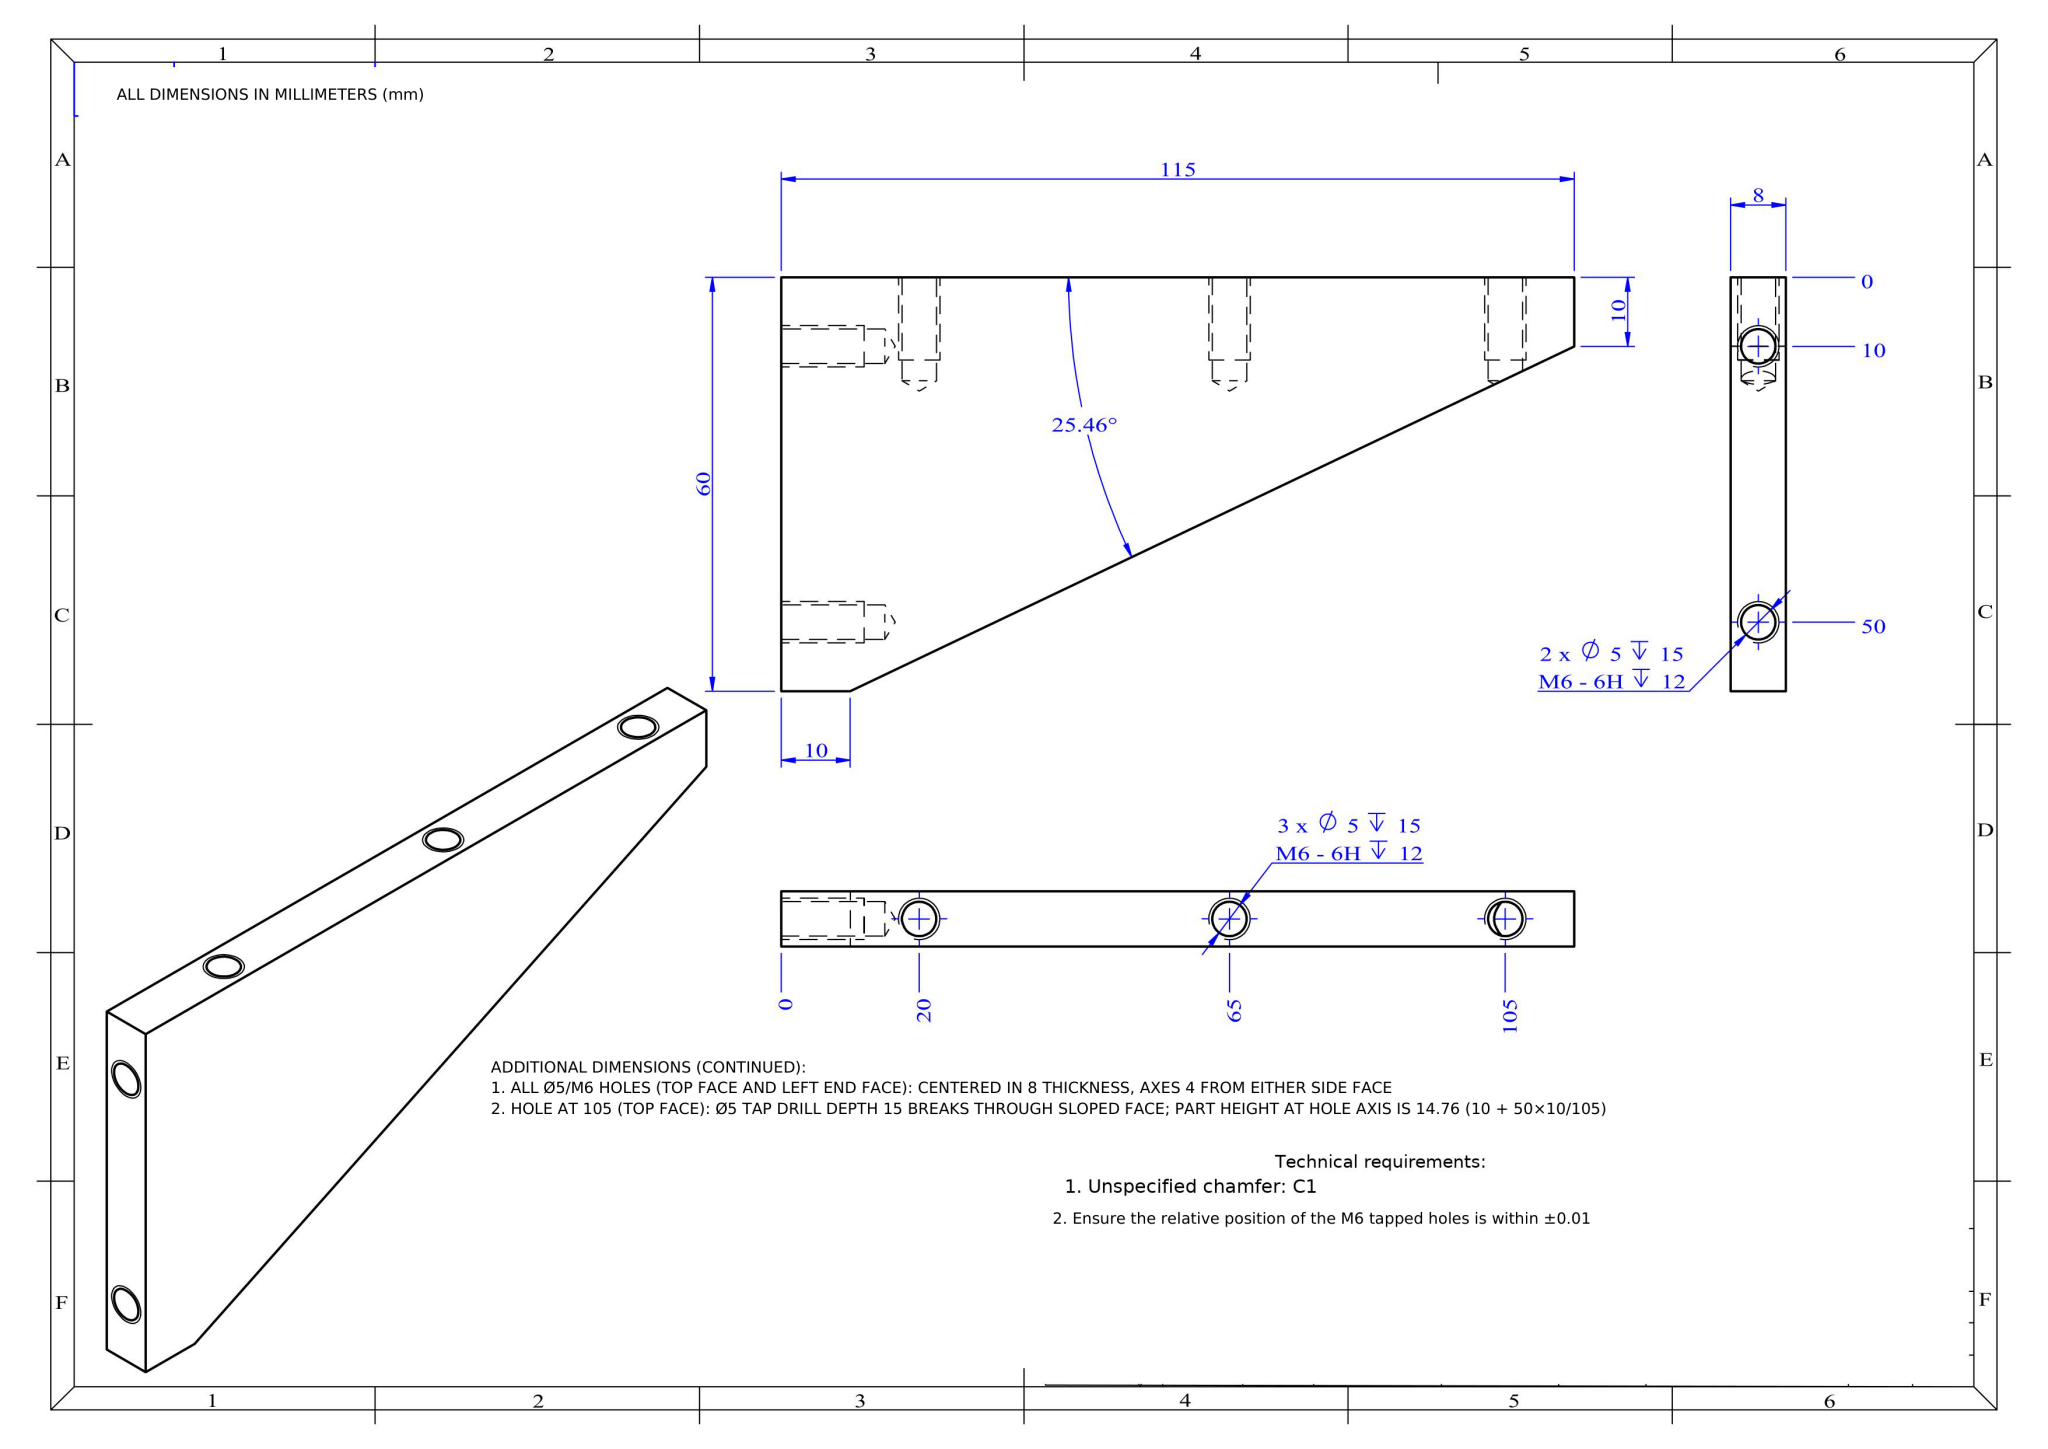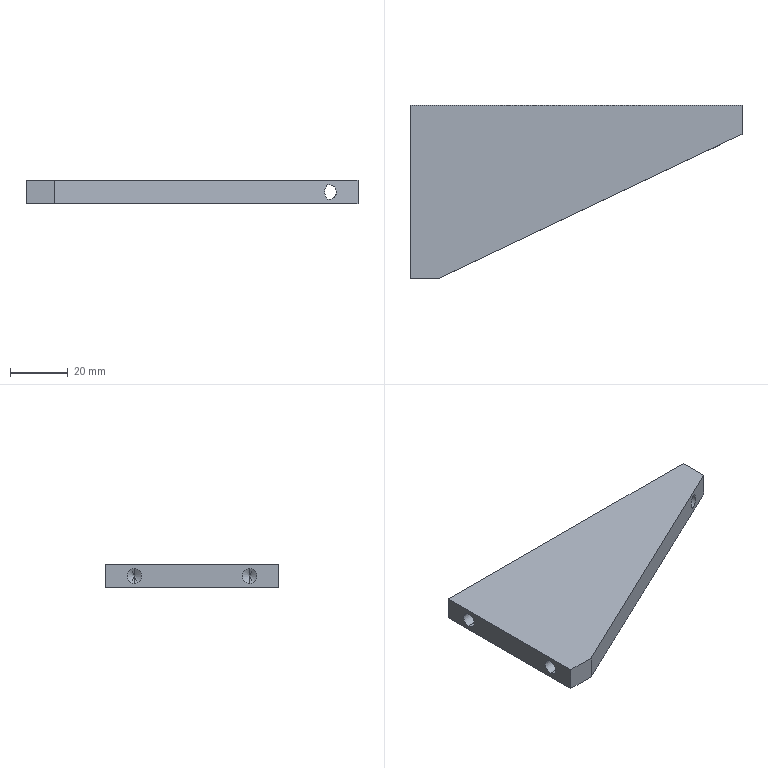Part | NX | mm | 1 solid | 26 faces | box 115 x 60 x 8 mm | volume 32694 mm3 | cylinder 10 | cone 9 | plane 7 | commonest cylinder face diameters 5 x10